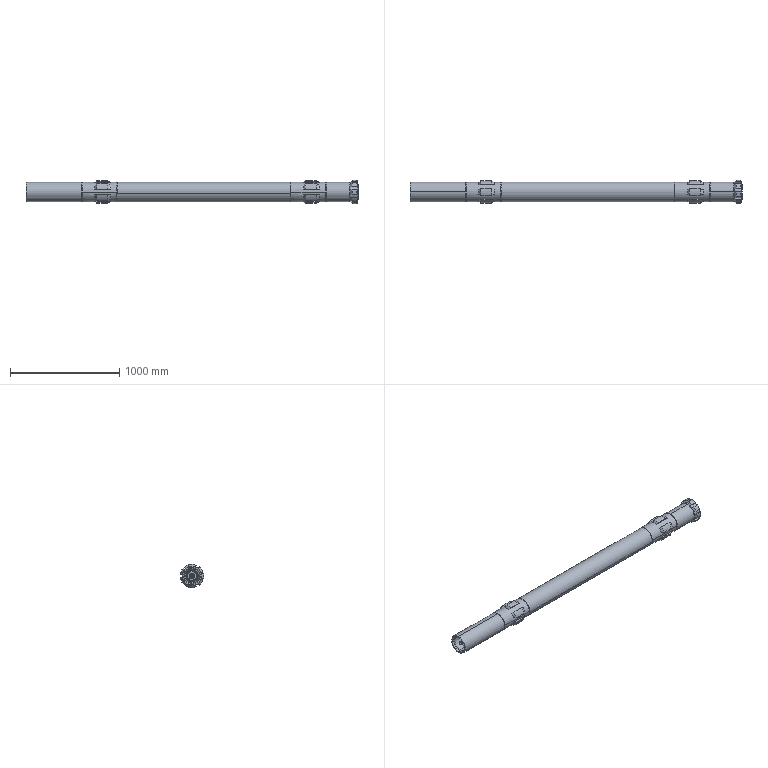Assembly | SolidWorks | mm | 55 component files | 55 solids | 1793 faces | box 3044.67 x 214.94 x 215.98 mm | volume 50933745 mm3 | cylinder 550 | plane 407 | cone 399 | torus 212 | sphere 202 | spline 23 | commonest cylinder face diameters 16 x24 20 x22 118 x21 96 x18 72 x18 6 x16 60 x14 210 x12
Bill of materials:
Adapter | 1 | Alloy Steel | Stepped, axially symmetric body with a central through bore. It has a long cylindrical section at one end, a larger-diameter central collar, and a short, smaller-diameter spigot at the other end. The collar has radial cross holes.
AdjustingShim | 2 | Alloy Steel | Thin, flat annular disc (washer-like ring) with a fairly wide radial face and a large central hole.
BearingPressSleeve1 | 1 | Alloy Steel | Short, thick-walled cylindrical ring or bushing with a through bore and an internal step (counterbore) at one end.
BearingSeat1 | 1 | Alloy Steel | Stepped, axially symmetric sleeve with a central raised collar between two cylindrical shoulders of different lengths. It has a through bore and a counterbore or step at one end.
BearingSleeve1 | 1 | Alloy Steel | Plain cylindrical sleeve with a stepped internal bore: a large-diameter bore from one end that narrows to a smaller through hole. Fine ring- or helix-like grooves are visible inside the larger bore.
BearingSpacer1 | 1 | Alloy Steel | Thin annular ring with a narrow radial wall and a small axial width; a band-like ring.
BearingSpacer2 | 1 | Alloy Steel | Thin annular ring with a narrow radial wall; similar to unnamed part but slightly wider axially.
CompressionRecoverySpring | 1 |  | Open-pitch helical coil of thin round wire, about 7 turns, with plain cut ends that are not closed or ground.
CompressionSpring | 1 |  | Open-pitch helical coil of thick round wire, about 5 turns, with a flat cut end face; its wire diameter is large relative to the coil diameter.
DampingSleeve | 1 | Polyurethane(11671) | Short, thin-walled cylindrical sleeve or ring with a large through bore, an outer chamfer at one end, and external circumferential grooves or steps on the outer diameter.
deep groove ball bearings gb | 2 |  | Annular assembly-like solid: an outer ring and an inner ring with about 13 spherical balls in the annular gap between them. It resembles a radial ball bearing.
FishingBody | 1 | Alloy Steel | Elongated tubular sleeve with a through bore. It has a larger-diameter section at one end, a reduced-diameter middle section with long axial slots that have rounded ends, a narrow band carrying small radial holes, and a slightly larger, chamfered section at the other end.
FishingSpearhead | 1 | Alloy Steel | Turned pin with a conical pointed end, stepped and tapered shank, a collar, and a slotted fork (clevis-like) end with a transverse through-hole across both prongs.
GB_T301-1995[ThrustBallBearing[51000]51305] | 1 |  | Thrust-ball-bearing-like assembly: two flat annular washers with a single ring of balls held between them.
GB_T301-1995[ThrustBallBearing[51000]51306] | 2 |  | Thrust-ball-bearing-like assembly very similar to the previous one: two annular washers separated by a ring of balls, with a slightly larger visible bore.
GuideSleeve | 1 | Alloy Steel | Thin-walled cylindrical sleeve with a short, slightly larger flange or step at one end.
HangingJoint | 1 | Alloy Steel | Hollow stepped cylindrical body with a raised collar, a waisted section, and a transverse through-hole, plus a stepped axial bore.
HangingRing | 1 | Alloy Steel | Flat annular ring or washer with chamfered outer edges on both faces.
hex nuts-style normal-grades ab gb | 2 |  | Tall hexagonal nut-like body with a round through-bore and chamfered hex corners on both ends.
InnerTube | 1 | Alloy Steel | Long, thin-walled straight round tube with plain cut ends.
InnerTubeJoint | 1 | Alloy Steel | Cylindrical sleeve or plug with a slightly raised band near one end, an axial bore open at that end, and a closed opposite end with a small central conical dimple.
Mandrel1 | 1 | Alloy Steel | Stepped turned shaft with a single larger disc collar, a short stepped stub on one side, and a longer two-diameter shank on the other.
RetainingRing | 1 | Alloy Steel | Very thin, narrow flat ring with a rectangular cross-section.
SnapRingSeat | 1 | Alloy Steel | Thin-walled cylindrical sleeve with a chamfer at one end.
SpearheadSeat | 1 | Alloy Steel | Long, thin, stepped, rotationally symmetric pin. One end is a flat tang with a cross hole. Partway along is a larger cylindrical collar, and the other end has a short, faceted, rounded or tapered nose.
SpringPlate | 4 | Alloy Steel | Straight bar with a square-to-rectangular cross-section. One end is chamfered or angled. The other end has a small round through hole, a small rectangular notch in one edge, and a concave curved end face.
SpringSleeve | 1 | Alloy Steel | Hollow cylindrical sleeve with two outside diameters: a longer large-diameter section and a shorter reduced-diameter section. A through bore runs the full length.
ValveGland | 1 | Alloy Steel | Short, stepped, hollow bushing-like part. It has a chamfered end land, a groove, a raised flange ring, and a cylindrical body with one flat cut on its side. A central round through hole runs the full length.
WaterSeparatorBall | 2 |  | Plain solid sphere.
CenteringRing | 1 | Brass | Thin-walled cylindrical ring or band with chamfered outer edges. Eight inward lugs or keys are spaced evenly around the bore.
LowerCentralizer | 1 | Alloy Steel | Hollow, stepped, cylindrical connector-like body. A larger-diameter section carries six radial ribs with chamfered ends, and a smaller section tapers toward an open end.
OuterTube | 1 | Alloy Steel | Long, slender, hollow tube with a short reduced-diameter, slightly tapered spigot at one end.
SeatRing | 1 | Alloy Steel | Plain thin-walled cylindrical ring or band with small chamfered or rounded outer edges. It has no internal features.
SpringClipChamber | 1 | Alloy Steel | Hollow cylindrical tube with a short, smaller-diameter, slightly tapered spigot at one end. It is shorter and wider than the tube in unnamed part.
UpperCentralizer | 1 | Alloy Steel | Hollow, stepped, cylindrical body with six chamfered external ribs on the larger section and a tapered smaller nose.
DrillBit | 1 | Alloy Steel | Hollow cylindrical sleeve with an enlarged, slotted crown or castellated head at one end. The head's end face has a ring of small blind holes around a central bore.
LocatingPin | 1 | Alloy Steel | Solid round cylinder with a small chamfer on one end edge and a flat end face at the other.
LocatingSpring | 1 |  | Open helical coil of round wire with constant coil diameter and even pitch, about 7 turns, with plain cut ends.
RetainingRingSeatCenteringRing | 1 | Alloy Steel | Short thin-walled cylindrical ring with about ten evenly spaced axial ribs projecting inward from the bore, and a small chamfer on one outer end edge.
SnapRing | 1 | Plain Carbon Steel | Very thin-walled open cylindrical sleeve with a narrow axial gap along its full length. The side views appear slightly tapered or uneven.
spring pin slotted heavy duty1 gb | 5 |  | Hollow tubular pin with a lengthwise slot through the wall and chamfered or tapered ends at both ends.
SpringClipRubberRing | 1 | Silicon Rubber | Thin circular ring (torus-like) with a small, apparently round cross-section relative to its diameter; shape is consistent with an O-ring-style toroid.
SpringClipRubberRing | 1 | Silicone Rubber | Closed round ring (torus) with a small circular cross-section relative to its diameter.
Mates:
1. coincident | 216OuterTube-1 plane at (0, 0, 0) dir (0, 0, 1) | assembly plane at (0, 0, 0) dir (0, 0, 1)
2. coincident | 216OuterTube-1 plane at (0, 0, 0) dir (0, 1, 0) | assembly plane at (0, 0, 0) dir (0, 1, 0)
3. coincident | 216OuterTube-1 plane at (0, 0, 0) dir (1, 0, 0) | assembly plane at (0, 0, 0) dir (1, 0, 0)
4. concentric | LocatingPin-1 face at (103.504, -0.02324, -0.000417) dir (1, 0, 0) r 7.5 | LocatingSpring-1 sketch segment at (95.504, -0.02324, -0.000417) dir (-1, 0, 0) r 4.5
5. coincident | LocatingPin-1 face at (95.504, -0.02324, -0.000417) dir (-1, 0, 0) | LocatingSpring-1 sketch segment at (95.504, -0.02324, -0.000417) dir (-1, 0, 0) r 4.5
6. coincident | 216InnerTubeAssembly-1/SpearheadSeat-1 face at (103.504, 18.997, 0.3412) dir (-1, 0, 0) | LocatingPin-1 face at (103.504, -0.02324, -0.000417) dir (1, 0, 0)
7. concentric | 216InnerTubeAssembly-1/FishingSpearhead-2 face at (160.493, -0.02324, -0.000417) dir (1, 0, 0) r 18.5 | LocatingPin-1 face at (103.504, -0.02324, -0.000417) dir (1, 0, 0) r 7.5
8. concentric | 216InnerTubeAssembly-1/FishingSpearhead-2 face at (128.504, -24.019, -0.4314) dir (0, 0.9998, 0.01796) r 8 | spring pin slotted heavy duty1 gb-1 face at (128.504, -19.752, -0.3547) dir (0, -0.9998, -0.01796) r 0.5
9. concentric | 216InnerTubeAssembly-1/FishingBody-1 face at (468.091, -39.856, 47.292) dir (0, 0.01796, -0.9998) r 3 | assembly face at (468.091, -37.303, -94.864) dir (0, -0.01796, 0.9998) r 3
10. concentric | 216InnerTubeAssembly-1/FishingBody-1 face at (468.091, -39.856, 47.292) dir (0, 0.01796, -0.9998) r 3 | spring pin slotted heavy duty1 gb-5 face at (468.091, -39.443, 24.256) dir (0, -0.01796, 0.9998) r 0.5
11. coincident | SpringClipRubberRing-1 sketch segment at (491.919, 0, 0) dir (1, 0, 0) | assembly plane at (0, 0, 0) dir (0, 0, 1)
12. coincident | SpringClipRubberRing-2 sketch segment at (486.543, 0, 0) dir (1, 0, 0) | assembly plane at (0, 0, 0) dir (0, 0, 1)
13. coincident | 216InnerTubeAssembly-1/RetainingRing-1 edge at (2899.778, 0, 0) dir (-1, 0, 0) r 46.5 | SnapRing-1 face at (2899.778, 48.524, -0.05575) dir (-1, 0, 0)
14. concentric | 216InnerTubeAssembly-1/SnapRingSeat-1 face at (2966.278, 0, 0) dir (1, 0, 0) r 47.848 | SnapRing-1 face at (2955.359, 0, 0) dir (1, 0, 0) r 43.633
15. concentric | DrillBit-1 face at (2750.079, 0, 0) dir (-1, 0, 0) r 89 | RetainingRingSeatCenteringRing-1 face at (2876.078, 0, 0) dir (-1, 0, 0) r 64
16. concentric | 216OuterTube-1/LowerCentralizer-1 face at (2425.901, 0, 0) dir (-1, 0, 0) r 89 | DrillBit-1 face at (2750.079, 0, 0) dir (-1, 0, 0) r 89
17. coincident | 216OuterTube-1/LowerCentralizer-1 face at (2750.079, 0, 0) dir (1, 0, 0) | DrillBit-1 face at (2750.079, 0, 0) dir (-1, 0, 0)
18. coincident | 216InnerTubeAssembly plane at (-417.302, -10.894, -59.447) dir (0, 0, 1) | 216InnerTubeAssembly plane at (0, 0, 0) dir (0, 0, 1)
19. coincident | 216InnerTubeAssembly plane at (-417.302, -10.894, -59.447) dir (0, 1, 0) | 216InnerTubeAssembly plane at (0, 0, 0) dir (0, 1, 0)
20. coincident | 216InnerTubeAssembly plane at (-417.302, -10.894, -59.447) dir (1, 0, 0) | 216InnerTubeAssembly plane at (0, 0, 0) dir (1, 0, 0)
21. coincident | SpringSleeve-1 plane at (0, 0, 0) dir (0, 0, 1) | 216InnerTubeAssembly plane at (0, 0, 0) dir (0, 0, 1)
22. coincident | SpringSleeve-1 plane at (0, 0, 0) dir (0, 1, 0) | 216InnerTubeAssembly plane at (0, 0, 0) dir (0, 1, 0)
23. coincident | SpringSleeve-1 plane at (0, 0, 0) dir (1, 0, 0) | 216InnerTubeAssembly plane at (0, 0, 0) dir (1, 0, 0)
24. concentric | SpringSleeve-1 face at (0, 0, 0) dir (1, 0, 0) r 34.995 | FishingBody-1 face at (-50.007, 0, 0) dir (1, 0, 0) r 174.533
25. coincident | SpringSleeve-1 edge at (-50.007, 0, 0) dir (1, 0, 0) r 43 | FishingBody-1 face at (-50.007, 0.000643, 0) dir (-1, 0, 0)
26. concentric | FishingBody-1 face at (164.101, 0, 0) dir (1, 0, 0) r 45 | GuideSleeve-1 face at (216.508, 0, 0) dir (1, 0, 0) r 35
27. coincident | FishingBody-1 face at (179.993, 0.000643, 0) dir (1, 0, 0) | GuideSleeve-1 face at (179.993, 35, 0) dir (-1, 0, 0)
28. concentric | FishingBody-1 face at (164.101, 0, 0) dir (1, 0, 0) r 35 | Adapter-1 face at (335.856, 0, 0) dir (1, 0, 0) r 36.5
29. coincident | FishingBody-1 face at (250.993, 0.000643, 0) dir (1, 0, 0) | Adapter-1 face at (250.993, 44, 0) dir (-1, 0, 0)
30. concentric | Adapter-1 face at (335.856, 0, 0) dir (1, 0, 0) r 24 | HangingJoint-1 face at (431.481, 0, 0) dir (1, 0, 0) r 24.678
31. coincident | Adapter-1 face at (306.481, 44, 0) dir (1, 0, 0) | HangingJoint-1 face at (306.481, 35, 0) dir (-1, 0, 0)
32. concentric | HangingJoint-1 face at (431.481, 0, 0) dir (1, 0, 0) r 36 | HangingRing-1 face at (328.636, 0, 0) dir (1, 0, 0) r 36
33. coincident | Adapter-1 face at (306.481, 44, 0) dir (1, 0, 0) | HangingRing-1 face at (306.481, 36.5, 0) dir (-1, 0, 0)
34. distance | 216InnerTubeAssembly face at (391.481, 0, 0) dir (-1, 0, 0) | HangingJoint-1 face at (431.481, 32.5, 0) dir (1, 0, 0)
35. concentric | HangingJoint-1 face at (431.481, 0, 0) dir (1, 0, 0) r 33.5 | 216InnerTubeAssembly face at (386.521, 0, 0) dir (-1, 0, 0) r 18
36. concentric | 216InnerTubeAssembly face at (386.521, 0, 0) dir (-1, 0, 0) r 18 | AdjustingShim-1 face at (422.955, 0, 0) dir (-1, 0, 0) r 20.5
37. coincident | HangingJoint-1 face at (431.481, 32.5, 0) dir (1, 0, 0) | AdjustingShim-1 face at (431.481, 29, 0) dir (-1, 0, 0)
38. concentric | 216InnerTubeAssembly face at (386.521, 0, 0) dir (-1, 0, 0) r 18 | AdjustingShim-2 face at (425.955, 0, 0) dir (-1, 0, 0) r 20.5
39. coincident | AdjustingShim-1 face at (434.481, 29, 0) dir (1, 0, 0) | AdjustingShim-2 face at (434.481, 29, 0) dir (-1, 0, 0)
40. concentric | 216InnerTubeAssembly face at (386.521, 0, 0) dir (-1, 0, 0) r 18 | hex nuts-style normal-grades ab gb-2 face at (437.481, 0, 0) dir (1, 0, 0) r 17.5
41. coincident | AdjustingShim-2 face at (437.481, 29, 0) dir (1, 0, 0) | hex nuts-style normal-grades ab gb-2 face at (437.481, -27.5, -15.877) dir (-1, 0, 0)
42. coincident | 216InnerTubeAssembly face at (503.481, 15, 0) dir (1, 0, 0) | 216InnerTubeAssembly face at (503.481, -0.2194, 0) dir (-1, 0, 0)
43. concentric | 216InnerTubeAssembly face at (386.521, 0, 0) dir (-1, 0, 0) r 15 | 216InnerTubeAssembly face at (503.359, 0, 0) dir (-1, 0, 0) r 40
44. concentric | 216InnerTubeAssembly face at (386.521, 0, 0) dir (-1, 0, 0) r 15 | GB_T301-1995[ThrustBallBearing[51000]51306]-1 face at (562.18, 0, 0) dir (1, 0, 0) r 15
45. coincident | 216InnerTubeAssembly face at (509.803, -0.2194, 0) dir (1, 0, 0) | GB_T301-1995[ThrustBallBearing[51000]51306]-1 face at (541.18, -30, 0) dir (-1, 0, 0)
46. concentric | 216InnerTubeAssembly face at (386.521, 0, 0) dir (-1, 0, 0) r 15 | GB_T301-1995[ThrustBallBearing[51000]51306]-2 face at (583.18, 0, 0) dir (1, 0, 0) r 15
47. coincident | GB_T301-1995[ThrustBallBearing[51000]51306]-1 face at (562.18, -30, 0) dir (1, 0, 0) | GB_T301-1995[ThrustBallBearing[51000]51306]-2 face at (562.18, -30, 0) dir (-1, 0, 0)
48. concentric | 216InnerTubeAssembly face at (386.521, 0, 0) dir (-1, 0, 0) r 12.5 | 216InnerTubeAssembly face at (653.446, 0, 0) dir (1, 0, 0) r 16
49. coincident | GB_T301-1995[ThrustBallBearing[51000]51306]-2 face at (583.18, -30, 0) dir (1, 0, 0) | 216InnerTubeAssembly face at (577.332, 0, 0) dir (-1, 0, 0)
50. concentric | 216InnerTubeAssembly face at (386.521, 0, 0) dir (-1, 0, 0) r 12.5 | GB_T301-1995[ThrustBallBearing[51000]51305]-1 face at (652.18, 0, 0) dir (-1, 0, 0) r 12.5
51. coincident | 216InnerTubeAssembly face at (652.332, 0, 0) dir (1, 0, 0) | GB_T301-1995[ThrustBallBearing[51000]51305]-1 face at (652.18, 9.928, -24.03) dir (-1, 0, 0)
52. concentric | 216InnerTubeAssembly face at (386.521, 0, 0) dir (-1, 0, 0) r 12.5 | CompressionSpring-1 sketch segment at (670.18, 0, 0) dir (1, 0, 0) r 20
53. coincident | GB_T301-1995[ThrustBallBearing[51000]51305]-1 face at (670.18, 9.928, -24.03) dir (1, 0, 0) | CompressionSpring-1 sketch segment at (670.18, 0, 0) dir (1, 0, 0) r 20
54. concentric | 216InnerTubeAssembly face at (386.521, 0, 0) dir (-1, 0, 0) r 12.5 | hex nuts-style normal-grades ab gb-1 face at (736.481, 0, 0) dir (1, 0, 0) r 17.5
55. distance | 216InnerTubeAssembly face at (734.481, 0, 0) dir (1, 0, 0) | hex nuts-style normal-grades ab gb-1 face at (771.181, -27.5, -15.877) dir (1, 0, 0)
56. concentric | FishingBody-1 face at (145.993, 39.001, -48) dir (0, 0, 1) r 3 | SpringPlate-1 face at (145.993, 39.001, 10.001) dir (0, 0, -1) r 3.25
57. distance | SpringPlate-1 face at (162.99, 43.443, 10.001) dir (0, 0, 1) | FishingBody-1 face at (180.993, 48, 10.501) dir (0, 0, -1)
58. concentric | SpringSleeve-1 face at (0, 0, 0) dir (1, 0, 0) r 43 | SpearheadSeat-1 face at (238.24, 0, 0) dir (1, 0, 0) r 29
59. distance | SpearheadSeat-1 face at (-218.594, 10, -29) dir (0, 1, 0) | FishingSpearhead-2 face at (-310.038, 10.5, 22.614) dir (0, -1, 0)
60. concentric | SpearheadSeat-1 face at (-193.594, 29, 0) dir (0, -1, 0) r 9 | FishingSpearhead-2 face at (-193.594, -24.023, 0) dir (0, 1, 0) r 8
61. coincident | SpearheadSeat-1 plane at (-74.788, -99.987, 0) dir (0, 0, 1) | 216InnerTubeAssembly plane at (0, 0, 0) dir (0, 0, 1)
62. parallel | SpearheadSeat-1 plane at (-74.788, -99.987, 0) dir (0, 1, 0) | 216InnerTubeAssembly plane at (0, 0, 0) dir (0, 1, 0)
63. concentric | SpearheadSeat-1 face at (238.24, 0, 0) dir (1, 0, 0) r 19 | CompressionRecoverySpring-1 sketch segment at (-74.594, 0, 0) dir (-1, 0, 0) r 26.5
64. coincident | SpearheadSeat-1 face at (-74.594, 26.5, 0) dir (-1, 0, 0) | CompressionRecoverySpring-1 sketch segment at (-74.594, 0, 0) dir (-1, 0, 0) r 26.5
65. concentric | HangingJoint-1 face at (431.481, 0, 0) dir (1, 0, 0) r 33.5 | Mandrel1-1 face at (780.974, 0, 0) dir (1, 0, 0) r 18
66. coincident | hex nuts-style normal-grades ab gb-2 face at (472.181, -27.5, -15.877) dir (1, 0, 0) | Mandrel1-1 face at (472.181, 18, 0) dir (-1, 0, 0)
67. concentric | Mandrel1-1 face at (780.974, 0, 0) dir (1, 0, 0) r 15 | BearingSleeve1-1 face at (623.853, 0, 0) dir (1, 0, 0) r 48
68. coincident | Mandrel1-1 face at (504.181, 15, 0) dir (1, 0, 0) | BearingSleeve1-1 face at (504.181, 0, 0) dir (-1, 0, 0)
69. concentric | Mandrel1-1 face at (780.974, 0, 0) dir (1, 0, 0) r 15 | BearingSpacer1-1 face at (519.181, 0, 0) dir (-1, 0, 0) r 27.5
70. coincident | BearingSleeve1-1 edge at (519.181, 0, 0) dir (1, 0, 0) r 34 | BearingSpacer1-1 face at (519.181, 27.5, 0) dir (-1, 0, 0)
71. concentric | Mandrel1-1 face at (780.974, 0, 0) dir (1, 0, 0) r 15 | BearingPressSleeve1-1 face at (519.181, 0, 0) dir (-1, 0, 0) r 36
72. coincident | BearingSleeve1-1 edge at (519.181, 0, 0) dir (1, 0, 0) r 34 | BearingPressSleeve1-1 face at (519.181, 0, 0) dir (-1, 0, 0)
73. concentric | Mandrel1-1 face at (780.974, 0, 0) dir (1, 0, 0) r 15 | deep groove ball bearings gb-2 face at (520.469, 0, 0) dir (-1, 0, 0) r 13
74. coincident | BearingSpacer1-1 face at (525.18, 22.5, 0) dir (1, 0, 0) | deep groove ball bearings gb-2 face at (525.18, 12.997, -0.2564) dir (-1, 0, 0)
75. concentric | GB_T301-1995[ThrustBallBearing[51000]51306]-1 face at (562.18, 0, 0) dir (1, 0, 0) r 30 | Mandrel1-1 face at (780.974, 0, 0) dir (1, 0, 0) r 15
76. coincident | GB_T301-1995[ThrustBallBearing[51000]51306]-1 face at (541.18, -30, 0) dir (-1, 0, 0) | BearingPressSleeve1-1 face at (541.18, 0, 0) dir (1, 0, 0)
77. concentric | GB_T301-1995[ThrustBallBearing[51000]51306]-2 face at (583.18, 0, 0) dir (1, 0, 0) r 30 | Mandrel1-1 face at (780.974, 0, 0) dir (1, 0, 0) r 15
78. concentric | Mandrel1-1 face at (780.974, 0, 0) dir (1, 0, 0) r 15 | BearingSpacer2-1 face at (583.18, 0, 0) dir (-1, 0, 0) r 27.5
79. coincident | GB_T301-1995[ThrustBallBearing[51000]51306]-2 face at (583.18, -30, 0) dir (1, 0, 0) | BearingSpacer2-1 face at (583.18, 0, 0) dir (-1, 0, 0)
80. concentric | Mandrel1-1 face at (780.974, 0, 0) dir (1, 0, 0) r 15 | deep groove ball bearings gb-3 face at (585.469, 0, 0) dir (-1, 0, 0) r 13
81. coincident | BearingSpacer2-1 face at (590.18, 0, 0) dir (1, 0, 0) | deep groove ball bearings gb-3 face at (590.18, 13, 0) dir (-1, 0, 0)
82. concentric | Mandrel1-1 face at (780.974, 0, 0) dir (1, 0, 0) r 15 | BearingSeat1-1 face at (569.653, 0, 0) dir (-1, 0, 0) r 48
83. coincident | deep groove ball bearings gb-3 face at (598.18, 13, 0) dir (1, 0, 0) | BearingSeat1-1 face at (598.18, 27.223, 2.743) dir (-1, 0, 0)
84. concentric | hex nuts-style normal-grades ab gb-1 face at (736.481, 0, 0) dir (1, 0, 0) r 17.5 | Mandrel1-1 face at (780.974, 0, 0) dir (1, 0, 0) r 12.5
85. coincident | hex nuts-style normal-grades ab gb-1 face at (771.181, -27.5, -15.877) dir (1, 0, 0) | Mandrel1-1 face at (771.181, 0, 0) dir (1, 0, 0)
86. concentric | BearingSeat1-1 face at (569.653, 0, 0) dir (-1, 0, 0) r 36 | InnerTubeJoint-2 face at (792.884, 0, 0) dir (-1, 0, 0) r 48
87. coincident | BearingSeat1-1 face at (633.18, 35.819, 3.609) dir (1, 0, 0) | InnerTubeJoint-2 face at (633.18, 0.1738, 0) dir (-1, 0, 0)
88. coincident | GB_T301-1995[ThrustBallBearing[51000]51305]-1 face at (652.18, 9.928, -24.03) dir (-1, 0, 0) | BearingSeat1-1 edge at (652.18, 0, 0) dir (-1, 0, 0) r 28
89. tangent | InnerTubeJoint-2 face at (827.359, 0.1738, 0) dir (1, 0, 0) | WaterSeparatorBall-1 face at (838.359, 0.5061, 0.09537) dir (1, 0, 0) r 11
90. concentric | InnerTubeJoint-2 face at (792.884, 0, 0) dir (-1, 0, 0) r 20 | ValveGland-1 face at (870.348, 0, 0) dir (1, 0, 0) r 20
91. coincident | InnerTubeJoint-2 face at (841.18, 0, 0) dir (1, 0, 0) r 1558.855 | ValveGland-1 edge at (841.329, 0, 0) dir (1, 0, 0) r 22.5
92. concentric | InnerTubeJoint-2 face at (792.884, 0, 0) dir (-1, 0, 0) r 48 | InnerTube-1 face at (821.18, 0, 0) dir (-1, 0, 0) r 49.4
93. coincident | InnerTubeJoint-2 face at (821.18, 0.1738, 0) dir (1, 0, 0) | InnerTube-1 face at (821.18, 0, 0) dir (-1, 0, 0)
94. concentric | InnerTube-1 face at (821.18, 0, 0) dir (-1, 0, 0) r 49 | SnapRingSeat-1 face at (2521.651, 0, 0) dir (-1, 0, 0) r 51.5
95. coincident | InnerTube-1 face at (2526.18, 0, 0) dir (1, 0, 0) | SnapRingSeat-1 face at (2526.18, 0.4163, 0) dir (-1, 0, 0)
96. concentric | SnapRingSeat-1 face at (2521.651, 0, 0) dir (-1, 0, 0) r 51.5 | RetainingRing-1 face at (2571.18, 0, 0) dir (-1, 0, 0) r 49
97. coincident | InnerTube-1 face at (2571.18, 0, 0) dir (1, 0, 0) | RetainingRing-1 face at (2571.18, 49, 0) dir (-1, 0, 0)
98. concentric | SnapRingSeat-1 face at (2644.18, 0, 0) dir (1, 0, 0) r 47.848 | 216InnerTubeAssembly face at (1637.462, 0, 0) dir (1, 0, 0) r 43.633
99. concentric | HangingJoint-1 face at (431.481, 0, 0) dir (1, 0, 0) r 36 | DampingSleeve-1 face at (336.484, 0, 0) dir (-1, 0, 0) r 15
100. coincident | HangingJoint-1 face at (351.481, 13, 0) dir (-1, 0, 0) | DampingSleeve-1 face at (351.481, -0.1681, 0.01381) dir (1, 0, 0)
101. tangent | DampingSleeve-1 face at (336.481, 0, 0) dir (1, 0, 0) r 174.533 | WaterSeparatorBall-2 face at (336.808, 0.4599, 0.08071) dir (1, 0, 0) r 11
102. concentric | SpringClipChamber-1 face at (0, 0, 0) dir (-1, 0, 0) r 89 | UpperCentralizer-1 face at (512.901, 0, 0) dir (-1, 0, 0) r 89
103. coincident | SpringClipChamber-1 face at (514.079, 0, 0) dir (1, 0, 0) | UpperCentralizer-1 face at (514.079, 0, 0) dir (-1, 0, 0)
104. concentric | UpperCentralizer-1 face at (512.901, 0, 0) dir (-1, 0, 0) r 89 | OuterTube-1 face at (1865.481, 0, 0) dir (-1, 0, 0) r 89
105. coincident | SpringClipChamber-1 plane at (0, 0, 0) dir (0, 0, 1) | 216OuterTube plane at (0, 0, 0) dir (0, 0, 1)
106. coincident | SpringClipChamber-1 plane at (0, 0, 0) dir (0, 1, 0) | 216OuterTube plane at (0, 0, 0) dir (0, 1, 0)
107. coincident | SpringClipChamber-1 plane at (0, 0, 0) dir (1, 0, 0) | 216OuterTube plane at (0, 0, 0) dir (1, 0, 0)
108. coincident | UpperCentralizer-1 face at (837.079, 0, 0) dir (1, 0, 0) | OuterTube-1 face at (837.079, 0, 0) dir (-1, 0, 0)
109. coincident | UpperCentralizer-1 edge at (692.079, 0, 0) dir (-1, 0, 0) r 64.5 | SeatRing-1 face at (692.079, 59, 0) dir (1, 0, 0)
110. concentric | SpringClipChamber-1 face at (635.079, 0, 0) dir (1, 0, 0) r 61.087 | SeatRing-1 face at (693.259, 0, 0) dir (1, 0, 0) r 64.5
111. coincident | LowerCentralizer-1 face at (2605.079, 0, 0) dir (-1, 0, 0) | CenteringRing-1 face at (2605.079, 0, 0) dir (1, 0, 0)
112. concentric | LowerCentralizer-1 face at (2425.901, 0, 0) dir (-1, 0, 0) r 89 | CenteringRing-1 face at (2591.223, 0, 0) dir (1, 0, 0) r 64
113. concentric | OuterTube-1 face at (1865.481, 0, 0) dir (-1, 0, 0) r 89 | LowerCentralizer-1 face at (2425.901, 0, 0) dir (-1, 0, 0) r 89
114. coincident | OuterTube-1 face at (2427.079, 0, 0) dir (1, 0, 0) | LowerCentralizer-1 face at (2427.079, 0, 0) dir (-1, 0, 0)